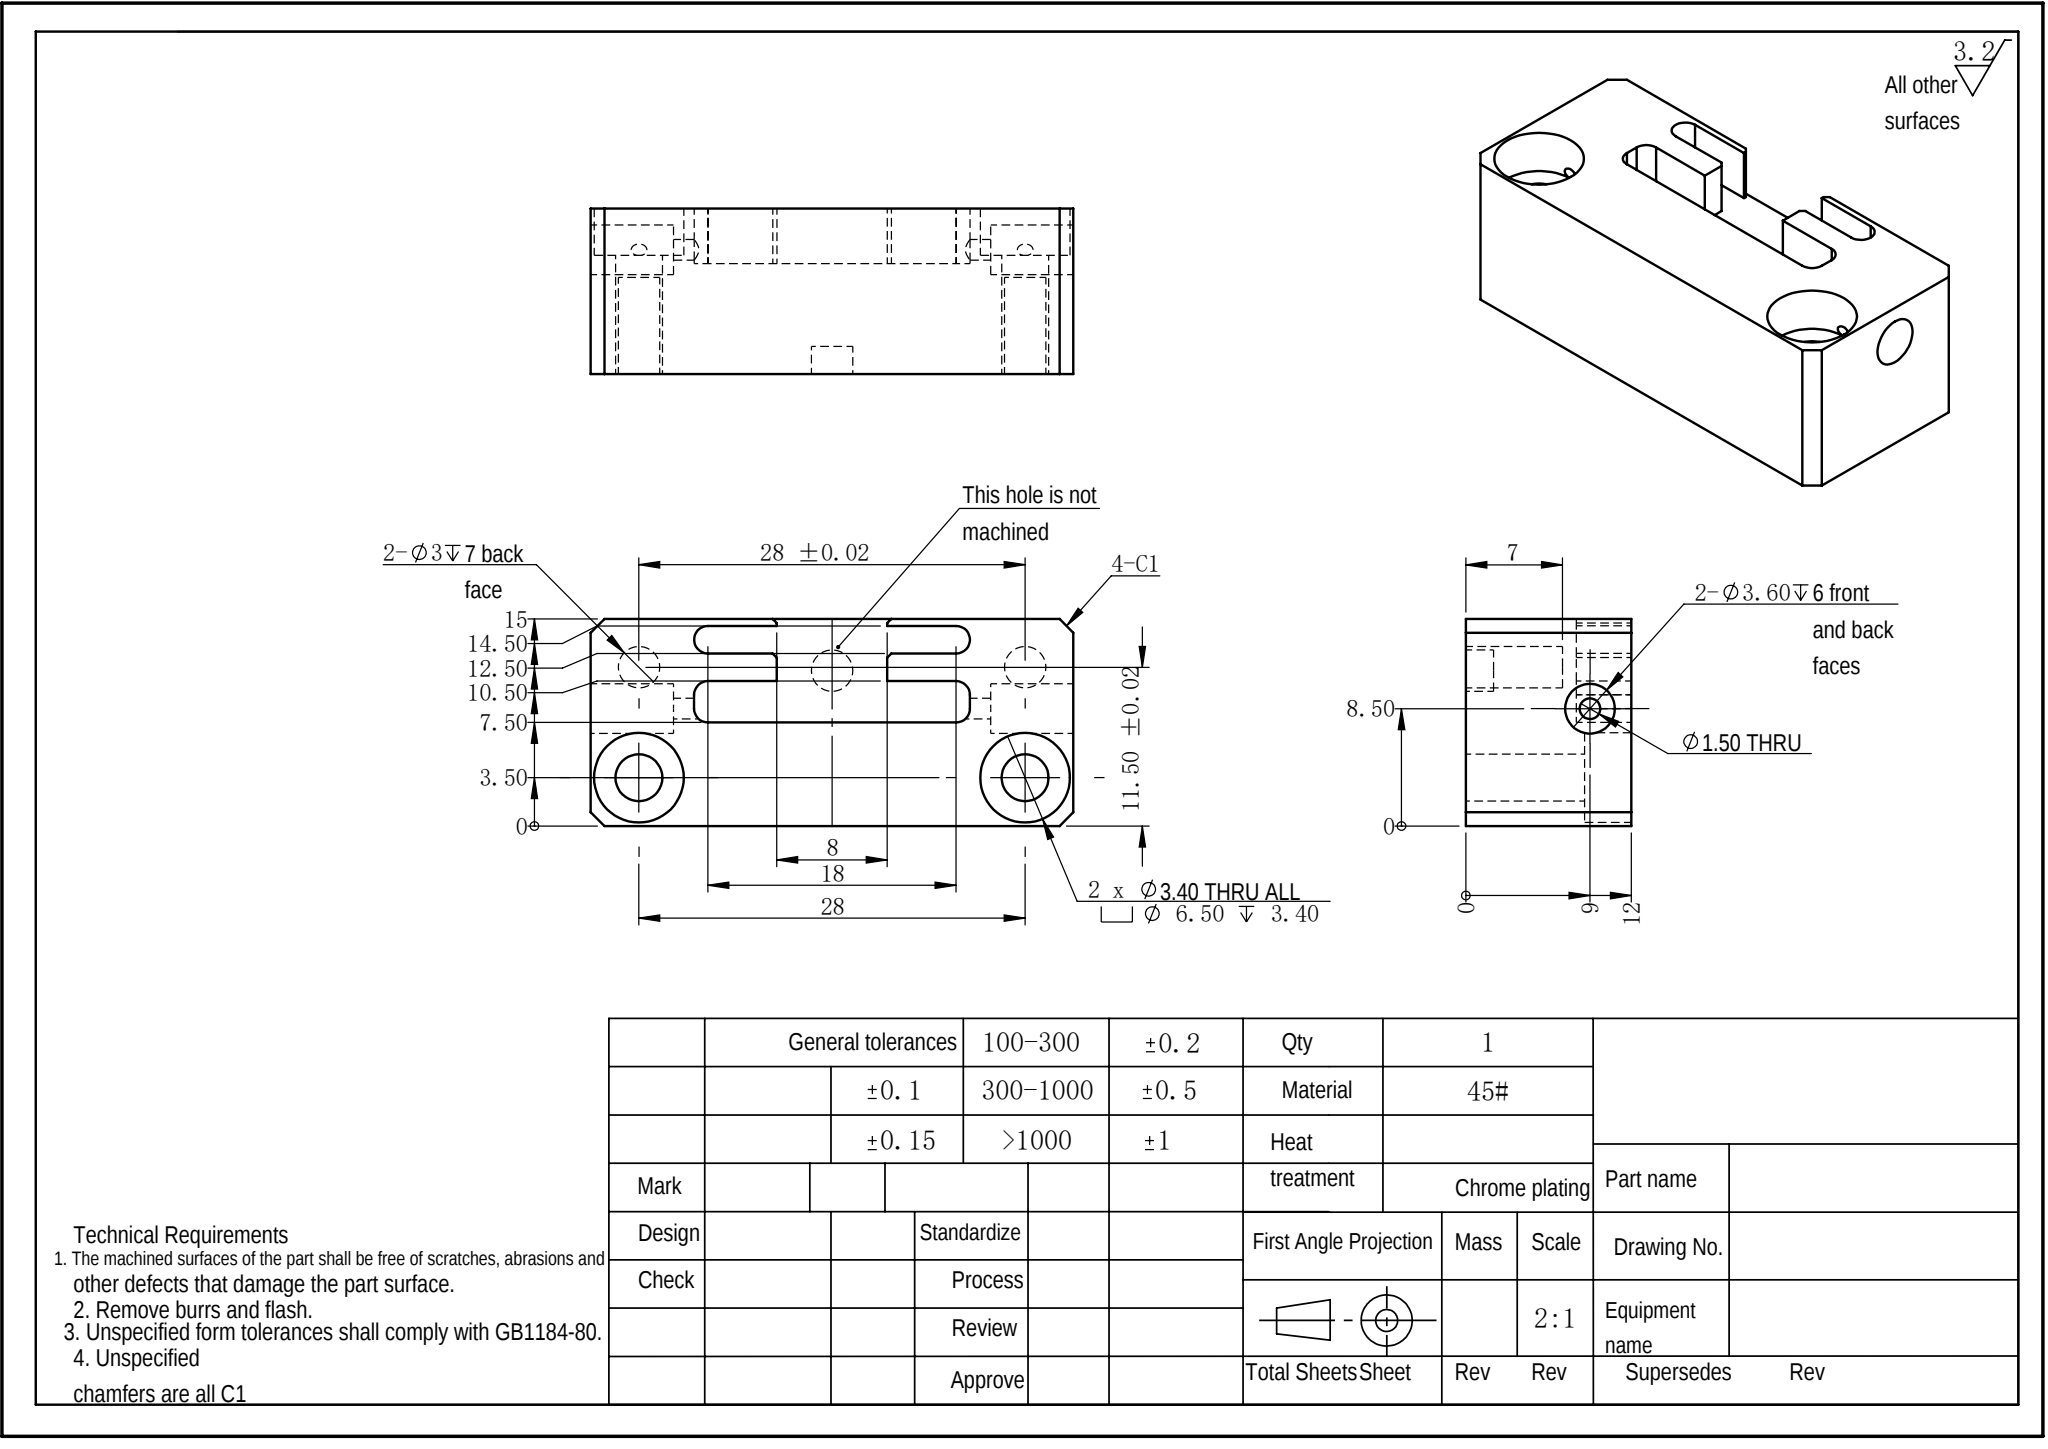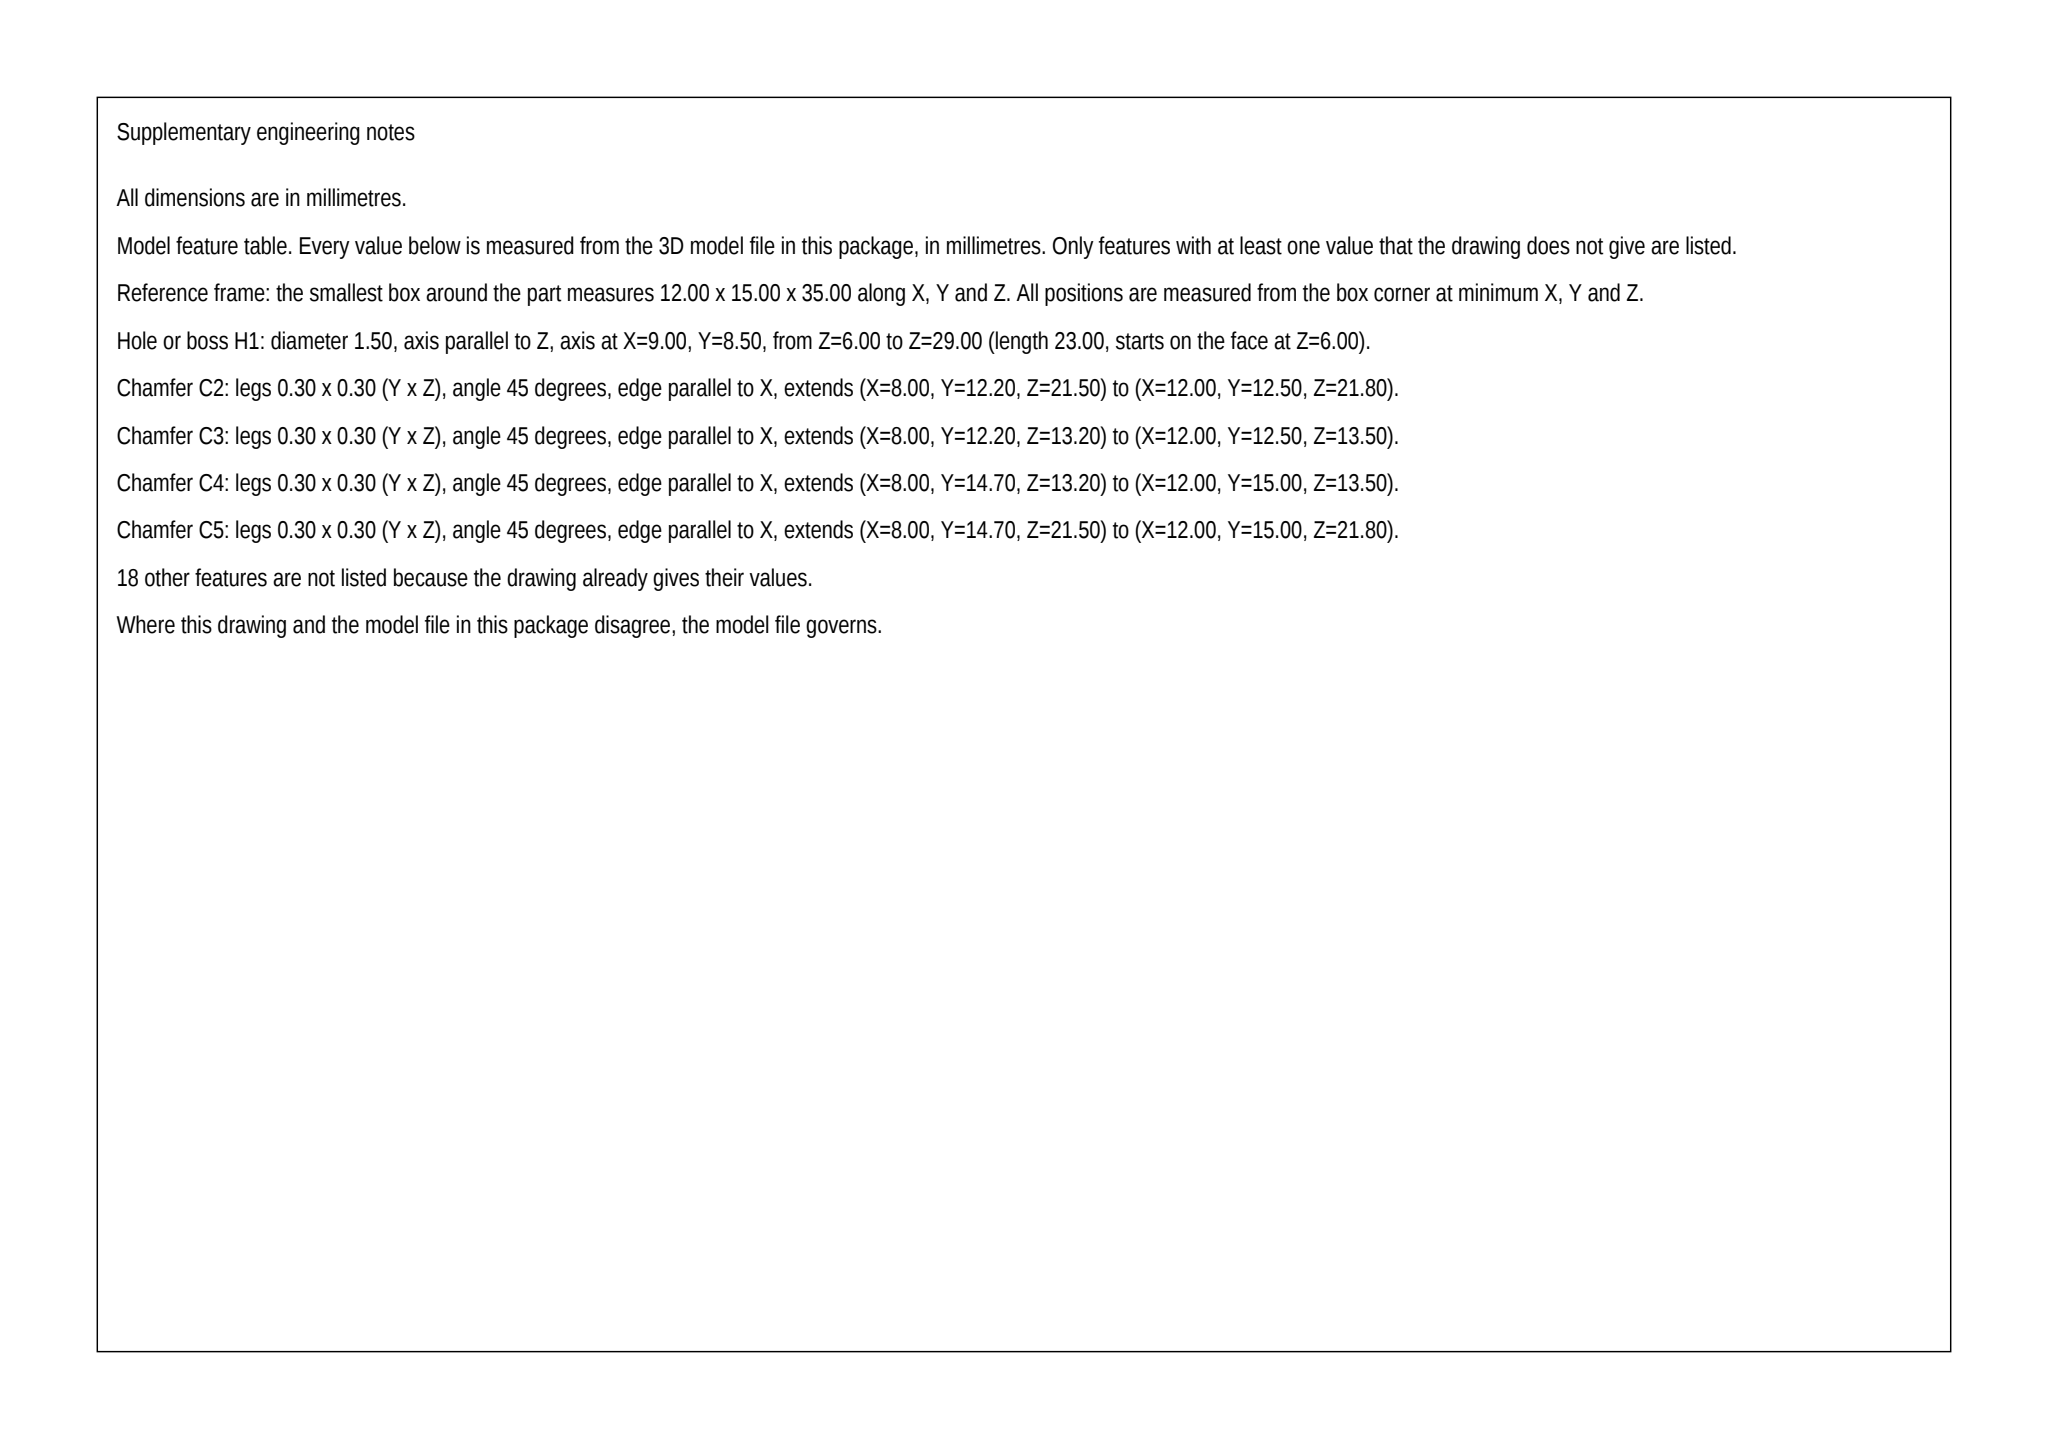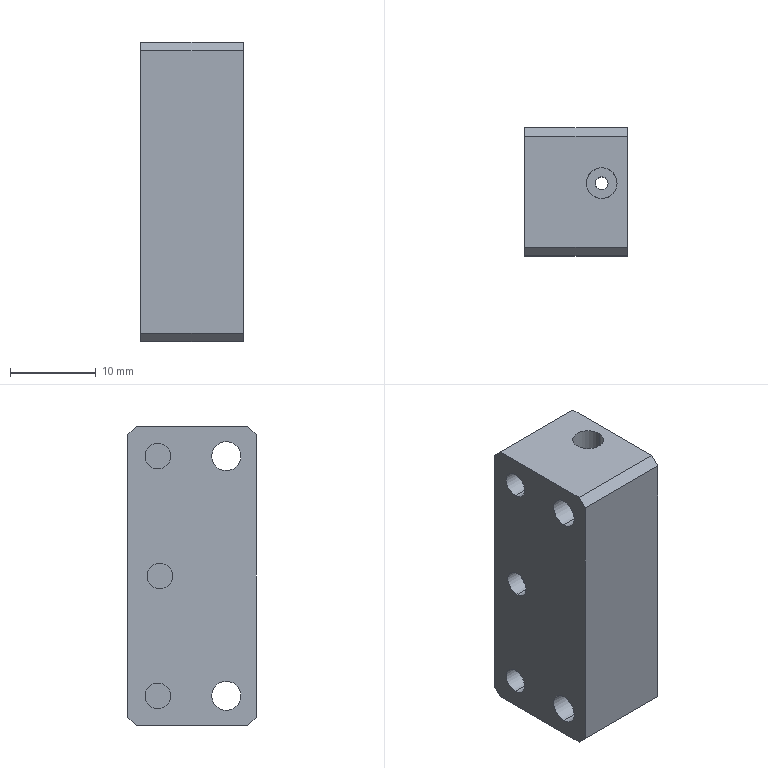Part | SolidWorks | mm | 1 solid | 64 faces | box 12 x 15 x 35 mm | volume 5180 mm3 | plane 35 | cylinder 29 | commonest cylinder face diameters 2 x7 3 x6 3.6 x4 3.4 x4 6.5 x4 1.5 x4
Drawing notes:
OVERALL LG 35 | from the solid: bbox_xyz z-extent = 35.0 (planes z=0 and z=35)
2X BACK SIDE END POCKET 6 LG X 5 DP (ONE EACH END) | from the solid: pocket walls at z=6.0 and z=29.0 (6 from each end, z=0/35); pocket floors plane x=7.0 (count 2) from back face x=12.0 -> 5 deep
build123d program:
from build123d import *

# Parameters (mm, degrees)
SKETCH1_W                                       = 12
SKETCH1_H                                       = 35
BOSS_EXTRUDE1_DEPTH                             = 15
SKETCH2_W                                       = 8
SKETCH2_H                                       = 8
CUT_EXTRUDE1_DEPTH                              = 7.5
CUT_EXTRUDE2_DEPTH                              = 4
M3_HEX_SOCKET_HEAD_CAP_SCREW_CBORE1_D           = 3.4
M3_HEX_SOCKET_HEAD_CAP_SCREW_CBORE1_CBORE_D     = 6.5
M3_HEX_SOCKET_HEAD_CAP_SCREW_CBORE1_CBORE_DEPTH = 3.4
CHAMFER1_SIZE                                   = 1
CUT_EXTRUDE3_REACH                              = 40.549
SKETCH6_R                                       = 0.75
SKETCH11_R                                      = 1.8
CUT_EXTRUDE6_DEPTH                              = 6
SKETCH14_R                                      = 1.5
CUT_EXTRUDE7_DEPTH                              = 7
LPATTERN1_COUNT                                 = 2
LPATTERN1_PITCH                                 = 5
CUT_EXTRUDE8_REACH                              = 27.986
SKETCH15_W                                      = 6.5
SKETCH15_H                                      = 2
FILLET1_R                                       = 1
SKETCH16_R                                      = 1.5
CUT_EXTRUDE9_DEPTH                              = 2
CHAMFER2_SIZE                                   = 0.3


with BuildPart() as part:
    # Sketch1 → Boss-Extrude1 (new body)
    with BuildSketch(Plane(origin=(0, 0, 0), x_dir=(1, 0, 0), z_dir=(0, 1, 0))):
        Rectangle(SKETCH1_W, SKETCH1_H)
    extrude(amount=BOSS_EXTRUDE1_DEPTH)

    # Sketch2 → Cut-Extrude1 (cut)
    with BuildSketch(Plane(origin=(0, 15, 0), x_dir=(1, 0, 0), z_dir=(0, 1, 0))):
        with Locations((6, 0)):
            Rectangle(SKETCH2_W, SKETCH2_H)
    extrude(amount=-CUT_EXTRUDE1_DEPTH, mode=Mode.SUBTRACT)

    # Sketch3 → Cut-Extrude2 (cut)
    with BuildSketch(Plane(origin=(6, 0, 0), x_dir=(0, 0, -1), z_dir=(1, 0, 0))):
        with BuildLine():
            Line((-9, 9.5), (-3, 9.5))
            ThreePointArc((-3, 9.5), (-2, 8.5), (-3, 7.5))
            Line((-3, 7.5), (-9, 7.5))
            ThreePointArc((-9, 7.5), (-10, 8.5), (-9, 9.5))
        make_face()
        with BuildLine():
            Line((9, 9.5), (3, 9.5))
            ThreePointArc((3, 9.5), (2, 8.5), (3, 7.5))
            Line((3, 7.5), (9, 7.5))
            ThreePointArc((9, 7.5), (10, 8.5), (9, 9.5))
        make_face()
    cut_extrude2 = extrude(amount=-CUT_EXTRUDE2_DEPTH, mode=Mode.SUBTRACT)

    # M3 Hex Socket Head Cap Screw CBORE1 (through all)
    with Locations(Plane(origin=(6, 0, 0), x_dir=(0, 0, -1), z_dir=(1, 0, 0))):
        with Locations((14, 3.5), (-14, 3.5)):
            CounterBoreHole(M3_HEX_SOCKET_HEAD_CAP_SCREW_CBORE1_D / 2, M3_HEX_SOCKET_HEAD_CAP_SCREW_CBORE1_CBORE_D / 2, M3_HEX_SOCKET_HEAD_CAP_SCREW_CBORE1_CBORE_DEPTH)

    # Chamfer1
    chamfer1_edges = [part.edges().sort_by_distance(p)[0] for p in [
        (0, 15, 17.5),
        (0, 0, 17.5),
        (0, 0, -17.5),
        (0, 15, -17.5),
    ]]
    chamfer(chamfer1_edges, length=CHAMFER1_SIZE)

    # Cut-Extrude3: up to this face of the body (flat: up to its plane)
    cut_extrude3_end = Plane(part.part.faces().sort_by_distance((0, 7.5, 17.5))[0])
    # Sketch6 → Cut-Extrude3 (cut, up to the picked face)
    with BuildSketch(Plane(origin=(0, 0, -17.5), x_dir=(-1, 0, 0), z_dir=(0, 0, -1)), mode=Mode.PRIVATE) as cut_extrude3_sk1:
        with Locations((-3, 8.5)):
            Circle(SKETCH6_R)
    cut_extrude3_tool1 = split(extrude(cut_extrude3_sk1.sketch, amount=-CUT_EXTRUDE3_REACH, mode=Mode.PRIVATE), bisect_by=cut_extrude3_end, keep=Keep.BOTH, mode=Mode.PRIVATE)
    add(cut_extrude3_tool1.solids().sort_by(Axis((3, 8.5, -17.5), (0, 0, 1)))[0], mode=Mode.SUBTRACT)

    # Sketch11 → Cut-Extrude6 (cut)
    with BuildSketch(Plane.XY.offset(17.5)):
        with Locations((3, 8.5)):
            Circle(SKETCH11_R)
    cut_extrude6 = extrude(amount=-CUT_EXTRUDE6_DEPTH, mode=Mode.SUBTRACT)

    # Mirror1: Cut-Extrude6 across plane
    add(cut_extrude6.mirror(Plane.XY), mode=Mode.SUBTRACT)

    # Sketch14 → Cut-Extrude7 (cut)
    with BuildSketch(Plane.ZY.offset(6)):
        with Locations((14, 11.5)):
            Circle(SKETCH14_R)
        with Locations(Location((-14, 11.5, 0), (0, 0, 180))):
            Circle(SKETCH14_R)
    extrude(amount=-CUT_EXTRUDE7_DEPTH, mode=Mode.SUBTRACT)

    # LPattern1: Cut-Extrude2 ×2
    with Locations(*[(0, i * LPATTERN1_PITCH, 0) for i in range(1, LPATTERN1_COUNT)]):
        add(cut_extrude2, mode=Mode.SUBTRACT)

    # Cut-Extrude8: up to this face of the body (flat: up to its plane)
    cut_extrude8_end = Plane(part.part.faces().sort_by_distance((2, 11.141, 0))[0])
    # Sketch15 → Cut-Extrude8 (cut, up to the picked face)
    with BuildSketch(Plane(origin=(6, 0, 0), x_dir=(0, 0, -1), z_dir=(1, 0, 0)), mode=Mode.PRIVATE) as cut_extrude8_sk1:
        with Locations((-6.75, 9.5)):
            Rectangle(SKETCH15_W, SKETCH15_H)
    cut_extrude8_tool1 = split(extrude(cut_extrude8_sk1.sketch, amount=-CUT_EXTRUDE8_REACH, mode=Mode.PRIVATE), bisect_by=cut_extrude8_end, keep=Keep.BOTH, mode=Mode.PRIVATE)
    # Sketch15 → Cut-Extrude8 (cut, up to the picked face)
    with BuildSketch(Plane(origin=(6, 0, 0), x_dir=(0, 0, -1), z_dir=(1, 0, 0)), mode=Mode.PRIVATE) as cut_extrude8_sk2:
        with Locations((6.75, 9.5)):
            Rectangle(SKETCH15_W, SKETCH15_H)
    cut_extrude8_tool2 = split(extrude(cut_extrude8_sk2.sketch, amount=-CUT_EXTRUDE8_REACH, mode=Mode.PRIVATE), bisect_by=cut_extrude8_end, keep=Keep.BOTH, mode=Mode.PRIVATE)
    add(cut_extrude8_tool1.solids().sort_by(Axis((6, 9.5, 6.75), (-1, 0, 0)))[0], mode=Mode.SUBTRACT)
    add(cut_extrude8_tool2.solids().sort_by(Axis((6, 9.5, -6.75), (-1, 0, 0)))[0], mode=Mode.SUBTRACT)

    # Fillet1
    fillet1_edges = [part.edges().sort_by_distance(p)[0] for p in [
        (4, 10.5, 10),
        (4, 10.5, -10),
    ]]
    fillet(fillet1_edges, radius=FILLET1_R)

    # Sketch16 → Cut-Extrude9 (cut)
    with BuildSketch(Plane.ZY.offset(6)):
        with Locations((0, 11.25)):
            Circle(SKETCH16_R)
    extrude(amount=-CUT_EXTRUDE9_DEPTH, mode=Mode.SUBTRACT)

    # Chamfer2
    chamfer2_edges = [part.edges().sort_by_distance(p)[0] for p in [
        (4, 12.5, 4),
        (4, 15, -4),
        (4, 12.5, -4),
        (4, 15, 4),
    ]]
    chamfer(chamfer2_edges, length=CHAMFER2_SIZE)


solid = part.part